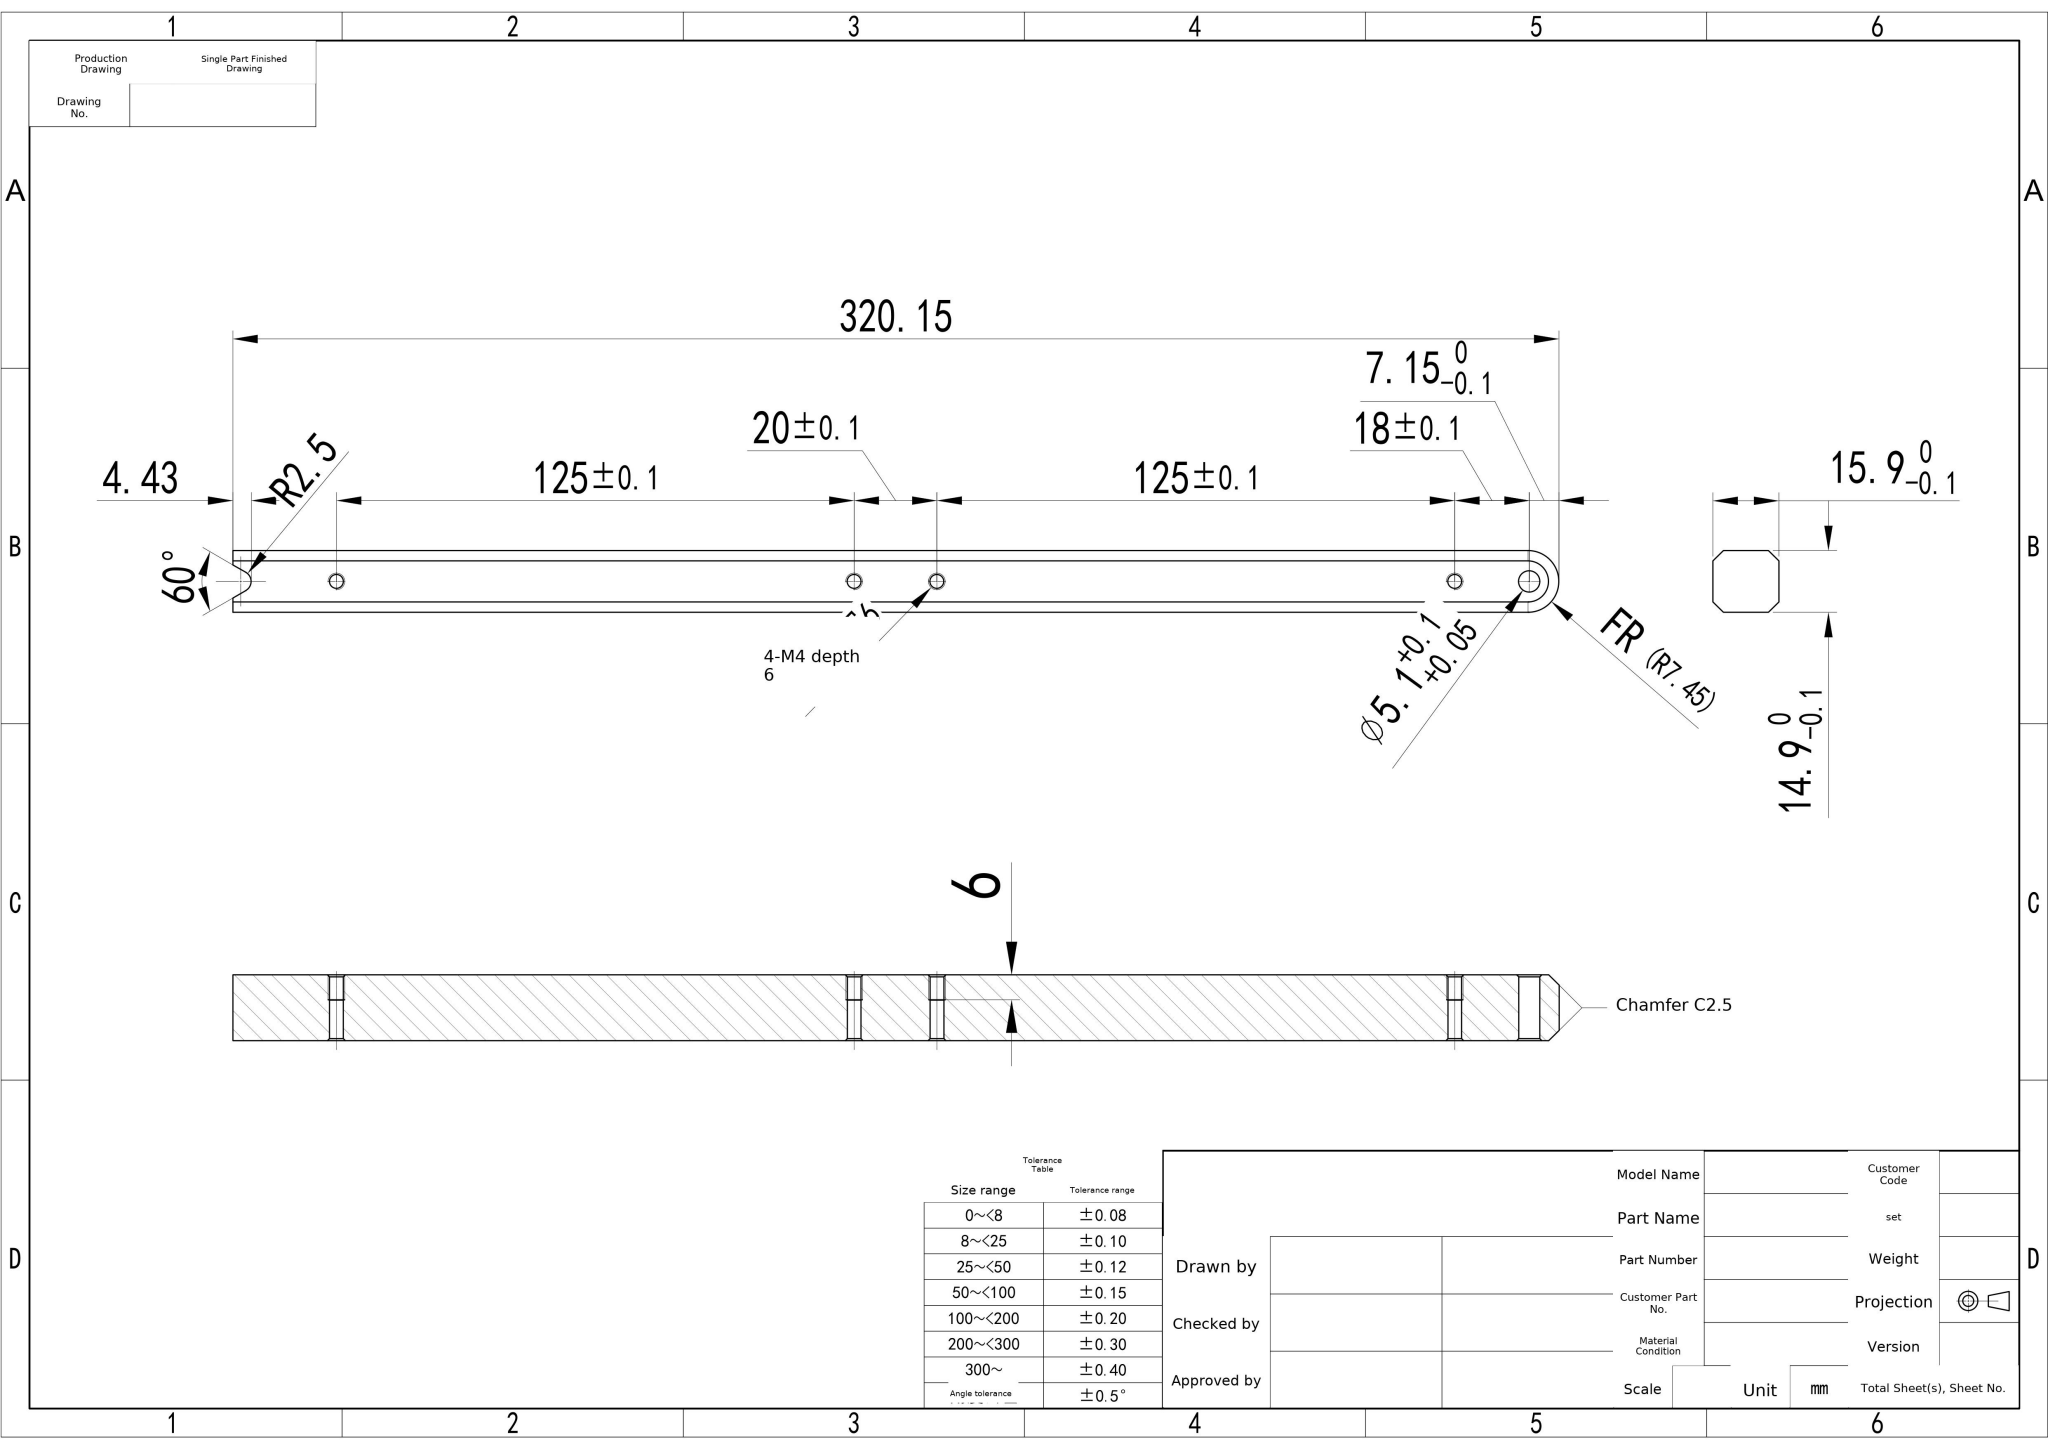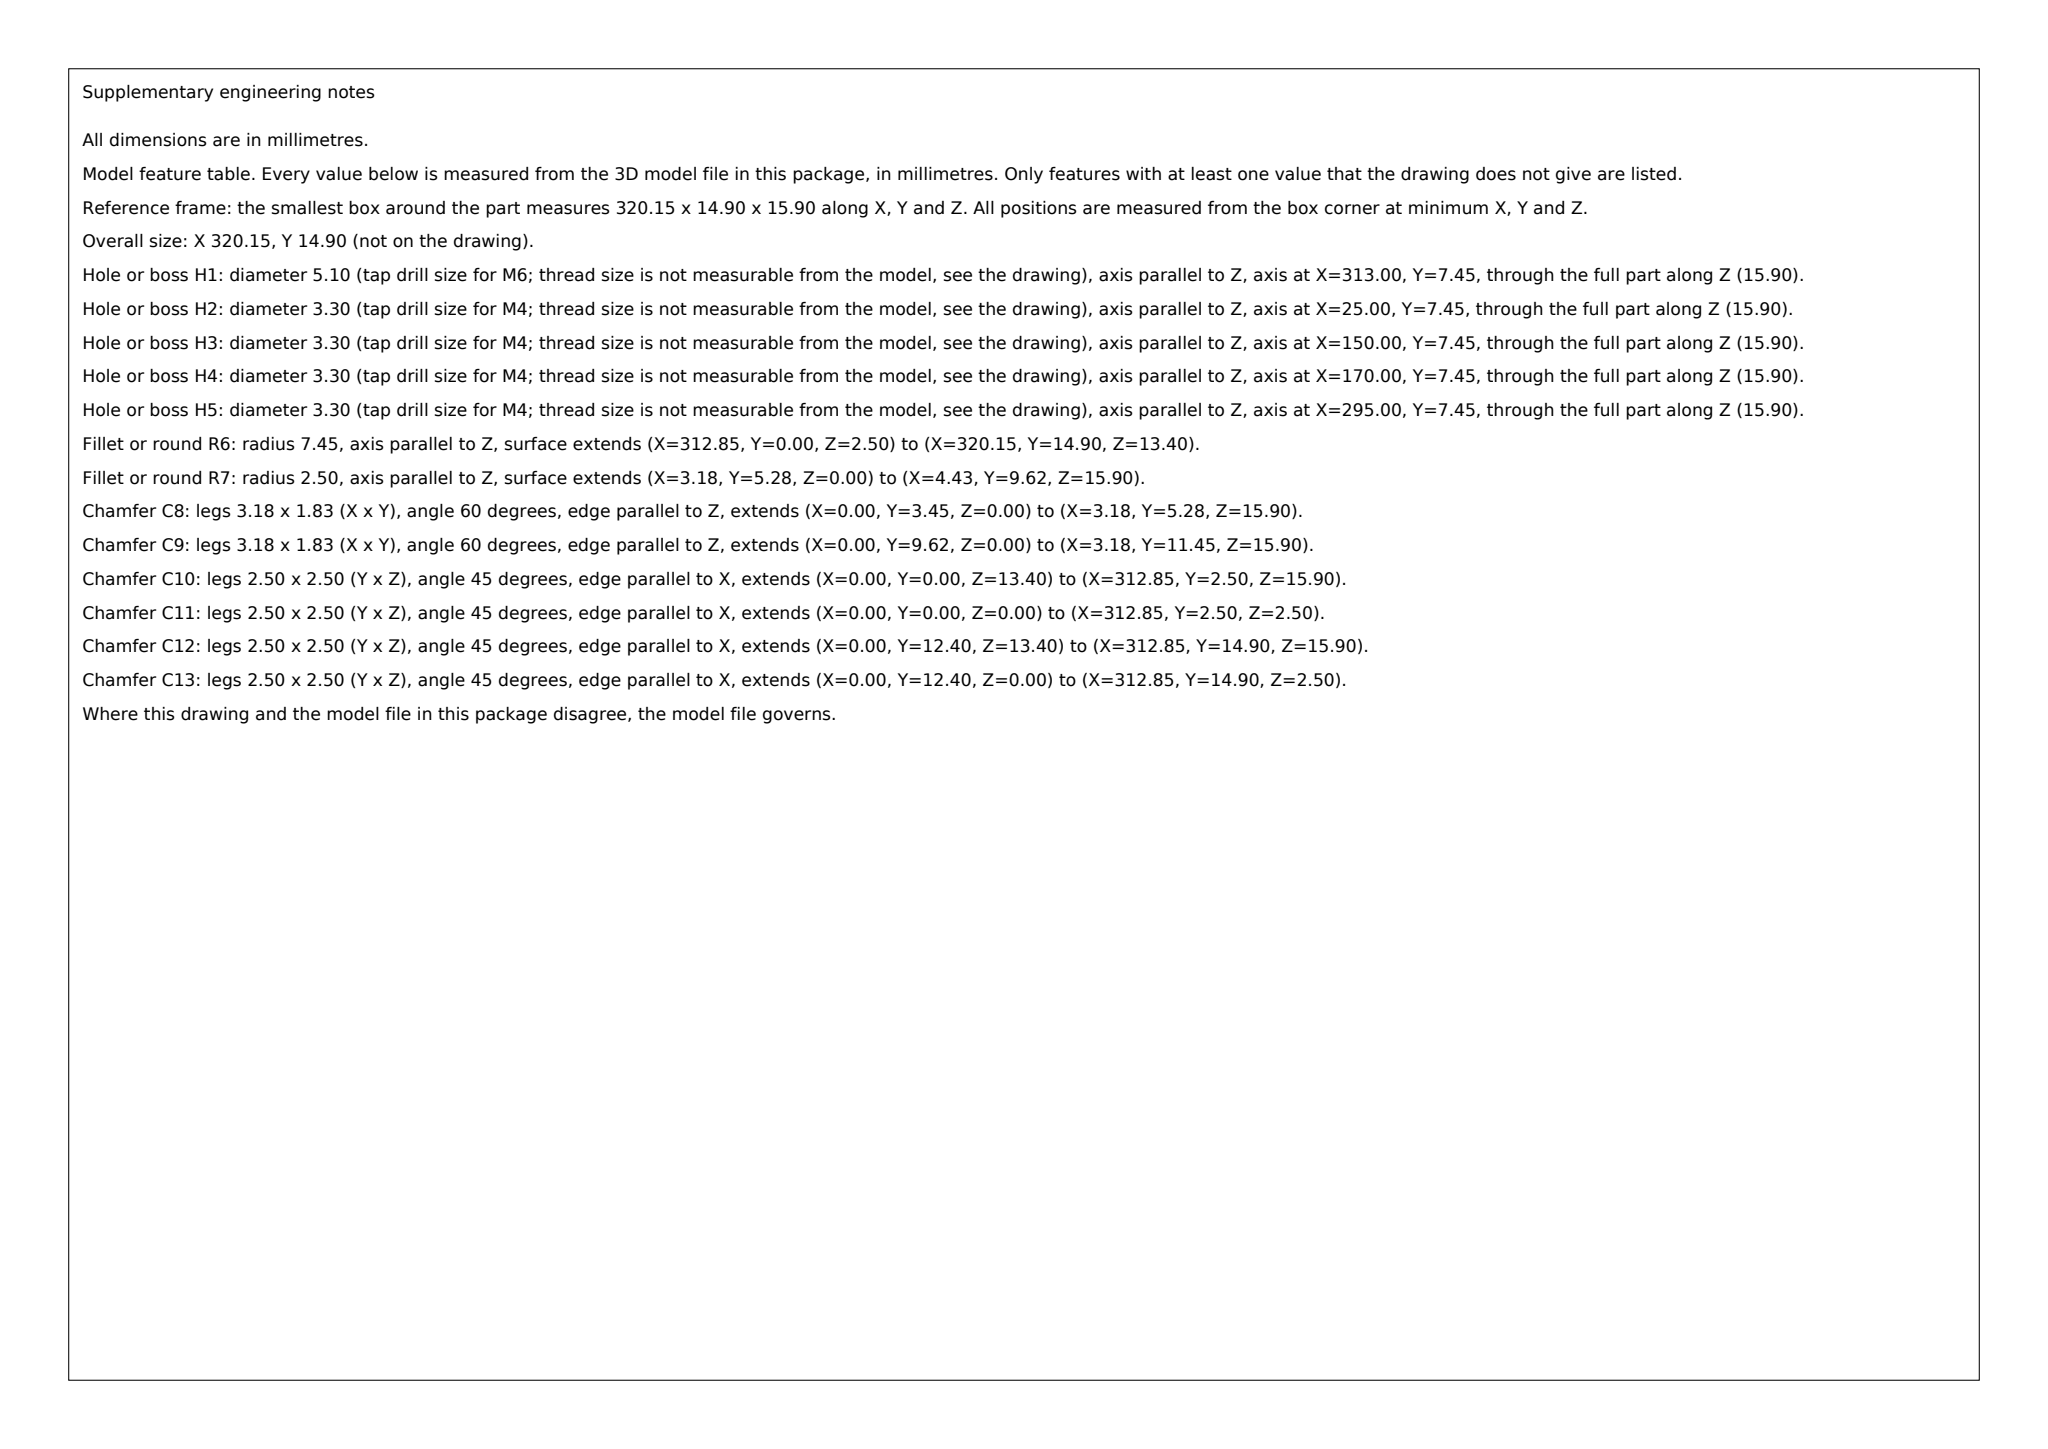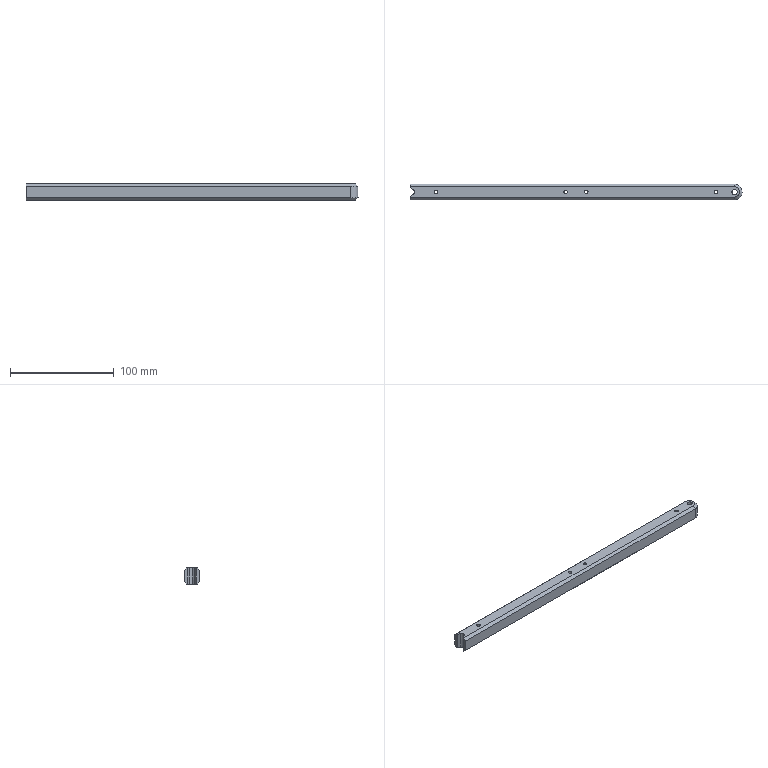Part | SolidWorks | mm | 1 solid | 28 faces | box 320.15 x 14.9 x 15.9 mm | volume 70204 mm3 | cylinder 14 | plane 12 | cone 2 | commonest cylinder face diameters 3.3 x8 14.9 x2 5.1 x2 5 x2